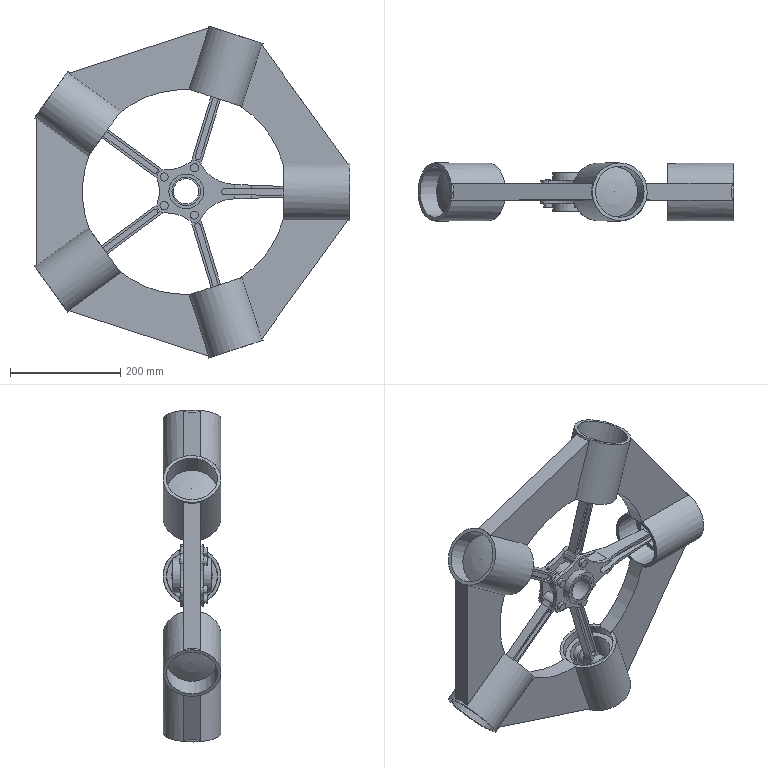Assembly | NX | mm | 60 component files | 60 solids | 652 faces | box 573.56 x 105 x 603.08 mm | volume 5426223 mm3 | plane 344 | cylinder 293 | torus 10 | sphere 5 | commonest cylinder face diameters 22 x30 92 x30 10 x28 84 x25 93 x25 36 x20 86 x20 48 x16
Bill of materials:
unnamed part 1 | 1 |  | Flat pentagon-shaped ring frame with a large round central opening. A short hollow cylindrical sleeve sits at each of the five corners.
unnamed part 2 | 4 |  | Plain straight round tube (hollow cylinder) with a moderately thick wall.
unnamed part 3 | 4 |  | Link with two cylindrical bosses of different sizes joined by a straight flat beam. Each boss has a through-bore, and the two bore axes are parallel.
unnamed part 4 | 4 |  | Solid stepped cylindrical pin: a long plain shank with a short head of larger diameter at one end.
unnamed part 5 | 5 |  | Piston-like cylindrical body with a flat or slightly domed top, several circumferential grooves near the top, one groove near the bottom, and a cross-bore through the side wall. The skirt is relieved (recessed) around the bore.
unnamed part 6 | 20 |  | Thin flat split ring with a rectangular cross-section and a small radial gap at one point on its circumference.
unnamed part 7 | 5 |  | Thick-walled round tube or spacer: a long cylinder with a small central through-bore.
unnamed part 8 | 5 |  | Thin-walled straight round tube of large diameter.
unnamed part 9 | 1 |  | Forked arm. At one end, two parallel flanges with lobed outlines sit on either side of a large hollow cylindrical hub. A tapering beam runs from the hub to a small hollow cylindrical boss at the other end.
unnamed part 10 | 1 |  | Straight round tube with a thin-to-moderate wall and a relatively short length compared with its diameter.
unnamed part 11 | 10 |  | Solid flanged pin or plug: a thin wide circular head with a rounded outer edge, plus a shorter cylindrical shank of smaller diameter.
Mates:
1. touch align | Rod_Bush_Upper 5 face | master_rod 1 face
2. touch align | master_rod 1 face | Rod_Bush_Upper 5 face
3. touch align | Rod_Bush_Upper 5 face | Radial_Engine 5 face
4. distance | Radial_Engine 5 face | master_rod 1 face
5. touch align | Piston_pin 5 face | Radial_Engine 5 face
6. distance | Piston_pin 5 face | Radial_Engine 5 face
7. touch align | Articulate_rod 3 face | master_rod 1 face
8. touch align | Articulate_rod 2 face | master_rod 1 face
9. touch align | Articulate_rod 1 face | master_rod 1 face
10. touch align | Articulate_rod 4 face | master_rod 1 face
11. touch align | Master_Rod_Bearing 1 face | master_rod 1 face
12. touch align | Master_Rod_Bearing 1 face | master_rod 1 face
13. touch align | Link_pin 1 face | master_rod 1 face
14. touch align | master_rod 1 face | Link_pin 3 face
15. touch align | master_rod 1 face | Link_pin 4 face
16. touch align | master_rod 1 face | Link_pin 2 face
17. touch align | Link_pin 1 face | master_rod 1 face
18. touch align | Link_pin 3 face | master_rod 1 face
19. touch align | Link_pin 4 face | master_rod 1 face
20. touch align | master_rod 1 face | Link_pin 2 face
21. touch align | Piston_Pin_Plug 10 face | Piston_pin 5 face
22. touch align | Piston_Pin_Plug 9 face | Piston_pin 5 face
23. touch align | Piston_Pin_Plug 9 face | Piston_pin 5 face
24. touch align | Piston_pin 5 face | Piston_Pin_Plug 10 face
25. touch align | Rod_Bush_Lower 2 face | Articulate_rod 2 face
26. touch align | Rod_Bush_Lower 4 face | Link_pin 3 face
27. touch align | Rod_Bush_Lower 3 face | Link_pin 1 face
28. touch align | Link_pin 2 face | Rod_Bush_Lower 1 face
29. touch align | Rod_Bush_Lower 4 face | Articulate_rod 1 face
30. touch align | Rod_Bush_Lower 3 face | Articulate_rod 4 face
31. touch align | Rod_Bush_Lower 2 face | Articulate_rod 2 face
32. touch align | Rod_Bush_Lower 1 face | Articulate_rod 3 face
33. touch align | Rod_Bush_Upper 1 face | Articulate_rod 3 face
34. touch align | Rod_Bush_Upper 2 face | Articulate_rod 2 face
35. touch align | Rod_Bush_Upper 3 face | Articulate_rod 1 face
36. touch align | Rod_Bush_Upper 4 face | Articulate_rod 4 face
37. touch align | Rod_Bush_Upper 4 face | Articulate_rod 4 face
38. touch align | Rod_Bush_Upper 3 face | Articulate_rod 1 face
39. touch align | Rod_Bush_Upper 2 face | Articulate_rod 2 face
40. touch align | Rod_Bush_Upper 1 face | Articulate_rod 3 face
41. touch align | Articulate_rod 4 face | master_rod 1 face
42. touch align | Articulate_rod 1 face | master_rod 1 face
43. touch align | Articulate_rod 2 face | master_rod 1 face
44. touch align | Articulate_rod 3 face | master_rod 1 face
45. touch align | Radial_Engine 1 face | Rod_Bush_Upper 1 face
46. touch align | Radial_Engine 2 face | Rod_Bush_Upper 2 face
47. touch align | Rod_Bush_Upper 3 face | Radial_Engine 3 face
48. touch align | Radial_Engine 4 face | Rod_Bush_Upper 4 face
49. distance | Articulate_rod 4 face | Radial_Engine 4 face
50. distance | Articulate_rod 2 face | Radial_Engine 2 face
51. distance | Radial_Engine 3 face | Articulate_rod 1 face
52. distance | Radial_Engine 1 face | Articulate_rod 3 face
53. touch align | Piston_pin 4 face | Radial_Engine 4 face
54. touch align | Piston_pin 3 face | Radial_Engine 3 face
55. touch align | Piston_pin 1 face | Radial_Engine 1 face
56. touch align | Piston_pin 2 face | Radial_Engine 2 face
57. distance | Piston_pin 1 face | Radial_Engine 1 face
58. distance | Piston_pin 2 face | Radial_Engine 2 face
59. distance | Piston_pin 3 face | Radial_Engine 3 face
60. distance | Piston_pin 4 face | Radial_Engine 4 face
61. touch align | Piston_Pin_Plug 1 face | Piston_pin 4 face
62. touch align | Piston_Pin_Plug 2 face | Piston_pin 4 face
63. touch align | Piston_Pin_Plug 4 face | Radial_Engine 3 face
64. touch align | Piston_Pin_Plug 3 face | Piston_pin 3 face
65. touch align | Piston_Pin_Plug 6 face | Piston_pin 2 face
66. touch align | Piston_Pin_Plug 7 face | Piston_pin 1 face
67. touch align | Piston_Pin_Plug 8 face | Radial_Engine 1 face
68. touch align | Piston_Pin_Plug 5 face | Piston_pin 2 face
69. touch align | Piston_Pin_Plug 8 face | Piston_pin 1 face
70. touch align | Piston_pin 1 face | Piston_Pin_Plug 7 face
71. touch align | Piston_Pin_Plug 6 face | Piston_pin 2 face
72. touch align | Piston_Pin_Plug 5 face | Piston_pin 2 face
73. touch align | Piston_Pin_Plug 4 face | Piston_pin 3 face
74. touch align | Piston_pin 3 face | Piston_Pin_Plug 3 face
75. touch align | Piston_Pin_Plug 1 face | Piston_pin 4 face
76. touch align | Piston_Pin_Plug 2 face | Piston_pin 4 face
77. fix | radial_engine_piston_Block 1 component
78. touch align | radial_engine_piston_Block 1 face | Radial_Engine 5 face
79. touch align | Piston_Ring 20 face | Radial_Engine 5 face
80. touch align | Piston_Ring 20 face | Radial_Engine 5 face
81. fix | assembly component
82. bond | Piston_Ring 20 component | assembly component
83. bond | Piston_Ring 19 component | assembly component
84. bond | Piston_Ring 18 component | assembly component
85. bond | Piston_Ring 17 component | assembly component
86. linear | assembly datumaxis | assembly cartesiancoordinatesystem | assembly cartesiancoordinatesystem | assembly cartesiancoordinatesystem | assembly cartesiancoordinatesystem
87. touch align | Piston_Ring 16 face | Radial_Engine 4 face
88. touch align | Piston_Ring 16 face | Radial_Engine 4 face
89. touch align | Piston_Ring 15 face | Radial_Engine 3 face
90. touch align | Piston_Ring 15 face | Radial_Engine 3 face
91. touch align | Piston_Ring 14 face | Radial_Engine 2 face
92. touch align | Piston_Ring 14 face | Radial_Engine 2 face
93. touch align | Piston_Ring 13 face | Radial_Engine 1 face
94. touch align | Piston_Ring 13 face | Radial_Engine 1 face
95. touch align | Radial_Engine 4 face | radial_engine_piston_Block 1 face
96. touch align | Radial_Engine 3 face | radial_engine_piston_Block 1 face
97. touch align | Radial_Engine 2 face | radial_engine_piston_Block 1 face
98. touch align | Radial_Engine 1 face | radial_engine_piston_Block 1 face
99. bond | radial_engine_piston_Block 1 component | assembly component
100. bond | Piston_Ring 16 component | assembly component
101. bond | Piston_Ring 12 component | assembly component
102. linear | assembly datumaxis | assembly cartesiancoordinatesystem | assembly cartesiancoordinatesystem | assembly cartesiancoordinatesystem | assembly cartesiancoordinatesystem
103. bond | Piston_Ring 11 component | assembly component
104. bond | Piston_Ring 10 component | assembly component
105. bond | Radial_Engine 2 component | assembly component
106. bond | Piston_Ring 14 component | assembly component
107. bond | Piston_Ring 9 component | assembly component
108. bond | Piston_Ring 8 component | assembly component
109. bond | Piston_Ring 7 component | assembly component
110. linear | assembly datumaxis | assembly cartesiancoordinatesystem | assembly cartesiancoordinatesystem | assembly cartesiancoordinatesystem | assembly cartesiancoordinatesystem
111. fix | assembly component
112. bond | Piston_Ring 13 component | assembly component
113. bond | Piston_Ring 6 component | assembly component
114. bond | Piston_Ring 5 component | assembly component
115. bond | Piston_Ring 4 component | assembly component
116. linear | assembly datumaxis | assembly cartesiancoordinatesystem | assembly cartesiancoordinatesystem | assembly cartesiancoordinatesystem | assembly cartesiancoordinatesystem
117. fix | assembly component
118. bond | Piston_Ring 15 component | assembly component
119. bond | Piston_Ring 3 component | assembly component
120. bond | Piston_Ring 2 component | assembly component
121. bond | Piston_Ring 1 component | assembly component
122. linear | assembly datumaxis | assembly cartesiancoordinatesystem | assembly cartesiancoordinatesystem | assembly cartesiancoordinatesystem | assembly cartesiancoordinatesystem